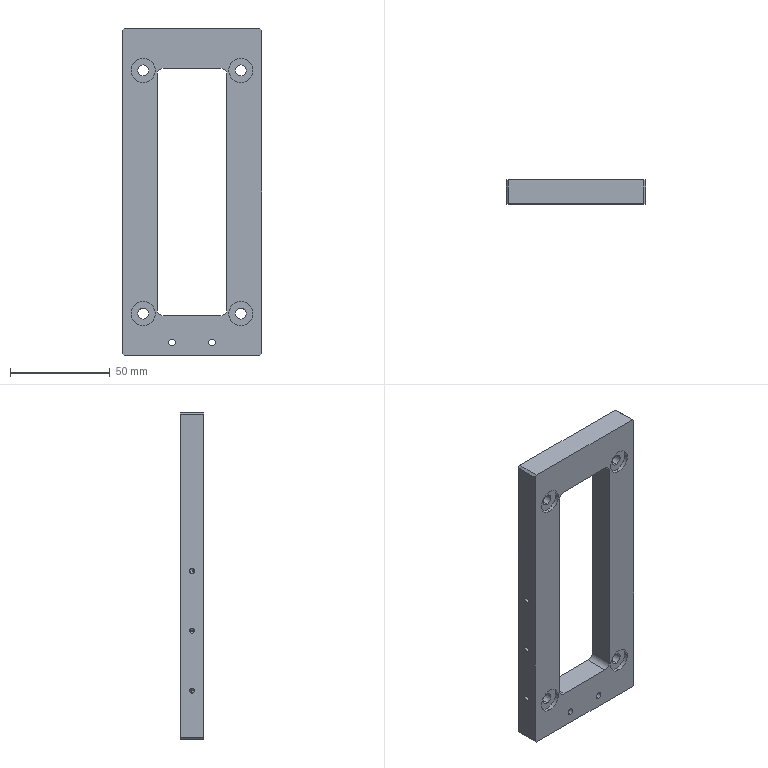Component | SolidWorks | F01AE00111-A2006-2 | 1 solid | 82 faces | box 70 x 12 x 164 mm | volume 82128 mm3 | cylinder 44 | plane 26 | cone 12 | commonest cylinder face diameters 2.5 x12 10 x8 5.5 x8 12 x8 3.3 x4 6 x4
build123d program:
from build123d import *

# Parameters (mm, degrees)
SKETCH1_2_W                                          = 164
SKETCH1_2_H                                          = 70
BOSS_EXTRUDE1_DEPTH                                  = 12
SKETCH2_R                                            = 1
CUT_EXTRUDE1_DEPTH                                   = 90.961
CHAMFER1_SIZE                                        = 1
SKETCH11_R                                           = 6
CUT_EXTRUDE4_DEPTH                                   = 2
HOLE_SIZE_ACCORDING_TO_THE_TYPE_1_OF_HEX_D           = 5.5
HOLE_SIZE_ACCORDING_TO_THE_TYPE_1_OF_HEX_CBORE_D     = 10
HOLE_SIZE_ACCORDING_TO_THE_TYPE_1_OF_HEX_CBORE_DEPTH = 5.7
M3_TAPPED_HOLE2_D                                    = 2.5
M3_TAPPED_HOLE2_DEPTH                                = 10
M3_TAPPED_HOLE2_TIP                                  = 0.7511
M3_TAPPED_HOLE3_D                                    = 2.5
M3_TAPPED_HOLE3_DEPTH                                = 10
M3_TAPPED_HOLE3_TIP                                  = 0.7511
M4_TAPPED_HOLE3_D                                    = 3.3
CUT_EXTRUDE5_DEPTH                                   = 20
SKETCH1_W                                            = 5.5
SKETCH1_H                                            = 4.6
IR_ELBOWRELIEF_DEPTH                                 = 1


with BuildPart() as part:
    # Sketch1_2 → Boss-Extrude1 (new body)
    with BuildSketch(Plane.XY):
        Rectangle(SKETCH1_2_W, SKETCH1_2_H)
    extrude(amount=BOSS_EXTRUDE1_DEPTH)

    # Sketch2 → Cut-Extrude1 (cut, through all)
    with BuildSketch(Plane.XY.offset(12)):
        with Locations((-61, 24.5)):
            Circle(SKETCH2_R)
        with Locations((-61, -24.5)):
            Circle(SKETCH2_R)
        with Locations((61, 24.5)):
            Circle(SKETCH2_R)
        with Locations((61, -24.5)):
            Circle(SKETCH2_R)
    extrude(amount=-CUT_EXTRUDE1_DEPTH, mode=Mode.SUBTRACT)

    # Chamfer1
    chamfer1_edges = [part.edges().sort_by_distance(p)[0] for p in [
        (82, -35, 6),
        (-82, -35, 6),
        (-82, 35, 6),
        (82, 35, 6),
    ]]
    chamfer(chamfer1_edges, length=CHAMFER1_SIZE)

    # Sketch11 → Cut-Extrude4 (cut)
    with BuildSketch(Plane(origin=(0, 0, 0), x_dir=(-1, 0, 0), z_dir=(0, 0, -1))):
        with Locations((-61, 24.5)):
            Circle(SKETCH11_R)
        with Locations((-61, -24.5)):
            Circle(SKETCH11_R)
        with Locations((61, 24.5)):
            Circle(SKETCH11_R)
        with Locations((61, -24.5)):
            Circle(SKETCH11_R)
    extrude(amount=-CUT_EXTRUDE4_DEPTH, mode=Mode.SUBTRACT)

    # Hole size according to the type 1 of hex (through all)
    with Locations(Plane.XY.offset(12)):
        with Locations((-61, 24.5), (61, 24.5), (61, -24.5), (-61, -24.5)):
            CounterBoreHole(HOLE_SIZE_ACCORDING_TO_THE_TYPE_1_OF_HEX_D / 2, HOLE_SIZE_ACCORDING_TO_THE_TYPE_1_OF_HEX_CBORE_D / 2, HOLE_SIZE_ACCORDING_TO_THE_TYPE_1_OF_HEX_CBORE_DEPTH)

    # M3 Tapped Hole2
    with Locations(Plane(origin=(0, -35, 0), x_dir=(-1, 0, 0), z_dir=(0, -1, 0))):
        with Locations((-57.5, -6), (-27.5, -6), (2.5, -6)):
            Hole(M3_TAPPED_HOLE2_D / 2, depth=M3_TAPPED_HOLE2_DEPTH)
            with Locations((0, 0, -(M3_TAPPED_HOLE2_DEPTH + M3_TAPPED_HOLE2_TIP / 2))):  # 118° drill point
                Cone(0, M3_TAPPED_HOLE2_D / 2, M3_TAPPED_HOLE2_TIP, mode=Mode.SUBTRACT)

    # M3 Tapped Hole3
    with Locations(Plane(origin=(0, 35, 0), x_dir=(1, 0, 0), z_dir=(0, 1, 0))):
        with Locations((-2.5, -6), (27.5, -6), (57.5, -6)):
            Hole(M3_TAPPED_HOLE3_D / 2, depth=M3_TAPPED_HOLE3_DEPTH)
            with Locations((0, 0, -(M3_TAPPED_HOLE3_DEPTH + M3_TAPPED_HOLE3_TIP / 2))):  # 118° drill point
                Cone(0, M3_TAPPED_HOLE3_D / 2, M3_TAPPED_HOLE3_TIP, mode=Mode.SUBTRACT)

    # M4 Tapped Hole3 (through all)
    with Locations(Plane.XY.offset(12)):
        with Locations((75.5, -10), (75.5, 10)):
            Hole(M4_TAPPED_HOLE3_D / 2)

    # Sketch37 → Cut-Extrude5 (cut)
    with BuildSketch(Plane.XY.offset(12)):
        with BuildLine():
            Line((-59, 17.5), (59, 17.5))
            ThreePointArc((59, 17.5), (61.121, 16.621), (62, 14.5))
            Line((62, 14.5), (62, -14.5))
            ThreePointArc((62, -14.5), (61.121, -16.621), (59, -17.5))
            Line((59, -17.5), (-59, -17.5))
            ThreePointArc((-59, -17.5), (-61.121, -16.621), (-62, -14.5))
            Line((-62, -14.5), (-62, 14.5))
            ThreePointArc((-62, 14.5), (-61.121, 16.621), (-59, 17.5))
        make_face()
    extrude(amount=-CUT_EXTRUDE5_DEPTH, mode=Mode.SUBTRACT)

    # Sketch1 → IR_ElbowRelief (cut, symmetric)
    with BuildSketch(Plane.XY.offset(12)):
        with Locations((46.475, 18.948)):
            Rectangle(SKETCH1_W, SKETCH1_H)
    extrude(amount=IR_ELBOWRELIEF_DEPTH, both=True, mode=Mode.SUBTRACT)


solid = part.part

# Placed as in the assembly
solid = solid.moved(Location((-109.352, 45.548, -272.475), (-90, 0, 90)))